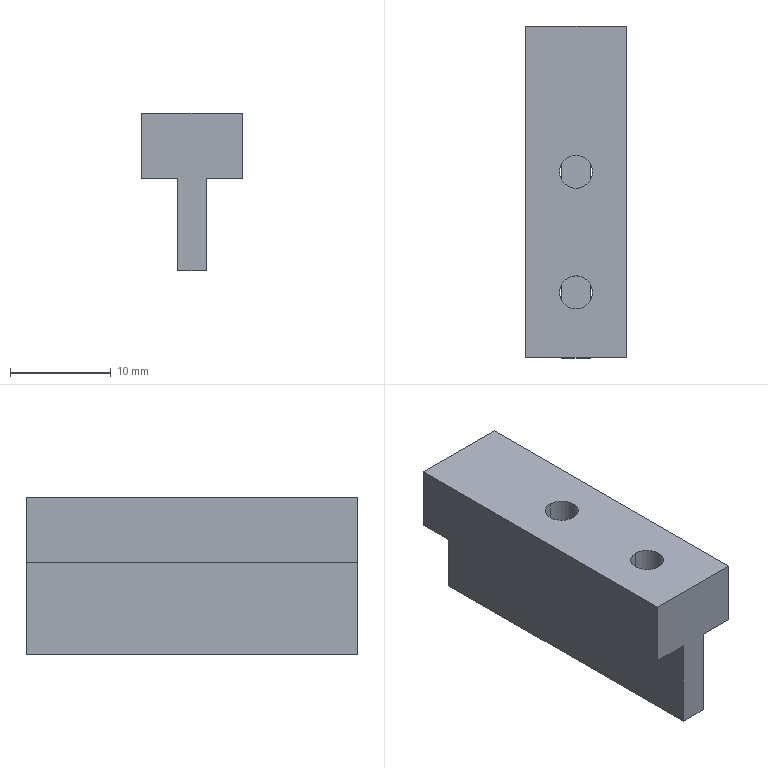Component | SolidWorks | 6G-TL06-X-AxisOrigin-1 | 1 solid | 16 faces | box 10 x 33 x 15.7 mm | volume 2884 mm3 | plane 12 | cylinder 4 | commonest cylinder face diameters 3.3 x4
build123d program:
from build123d import *

# Parameters (mm, degrees)
SKETCH1_W           = 33
SKETCH1_H           = 10
BOSS_EXTRUDE1_DEPTH = 6.5
M4_TAPPED_HOLE1_D   = 3.3
SKETCH7_W           = 33
SKETCH7_H           = 2.8
BOSS_EXTRUDE2_DEPTH = 9.2


with BuildPart() as part:
    # Sketch1 → Boss-Extrude1 (new body)
    with BuildSketch(Plane.XY):
        Rectangle(SKETCH1_W, SKETCH1_H)
    extrude(amount=-BOSS_EXTRUDE1_DEPTH)

    # M4 Tapped Hole1 (through all)
    with Locations(Plane(origin=(-10, 0, -6.5), x_dir=(-1, 0, 0), z_dir=(0, 0, -1))):
        with Locations((0, 0), (-12, 0)):
            Hole(M4_TAPPED_HOLE1_D / 2)

    # Sketch7 → Boss-Extrude2 (add)
    with BuildSketch(Plane(origin=(0, 0, -6.5), x_dir=(-1, 0, 0), z_dir=(0, 0, -1))):
        Rectangle(SKETCH7_W, SKETCH7_H)
    extrude(amount=BOSS_EXTRUDE2_DEPTH)


solid = part.part

# Placed as in the assembly
solid = solid.moved(Location((46, 333, -25), (0, 0, 90)))
STEP:
#1=COLOUR_RGB('',0.7922,0.8196,0.9333);
#2=FILL_AREA_STYLE_COLOUR('',#1);
#3=FILL_AREA_STYLE('',(#2));
#4=SURFACE_STYLE_FILL_AREA(#3);
#5=SURFACE_SIDE_STYLE('',(#4));
#6=SURFACE_STYLE_USAGE(.BOTH.,#5);
#7=PRESENTATION_STYLE_ASSIGNMENT((#6));
#8=CARTESIAN_POINT('',(1.811,12.781,-0.9843));
#9=VERTEX_POINT('',#8);
#10=CARTESIAN_POINT('',(1.811,12.652,-0.9843));
#11=VERTEX_POINT('',#10);
#12=CARTESIAN_POINT('',(1.811,12.717,-0.9843));
#13=DIRECTION('',(0.,-0.,-1.));
#14=DIRECTION('',(0.,-1.,0.));
#15=AXIS2_PLACEMENT_3D('',#12,#13,#14);
#16=CIRCLE('',#15,0.06496);
#17=EDGE_CURVE('',#9,#11,#16,.T.);
#18=ORIENTED_EDGE('',*,*,#17,.F.);
#19=CARTESIAN_POINT('',(1.811,12.781,-1.24));
#20=VERTEX_POINT('',#19);
#21=CARTESIAN_POINT('',(1.811,12.781,-1.24));
#22=DIRECTION('',(0.,-0.,-1.));
#23=VECTOR('',#22,39.37);
#24=LINE('',#21,#23);
#25=EDGE_CURVE('',#9,#20,#24,.T.);
#26=ORIENTED_EDGE('',*,*,#25,.T.);
#27=CARTESIAN_POINT('',(1.866,12.751,-1.24));
#28=VERTEX_POINT('',#27);
#29=CARTESIAN_POINT('',(1.811,12.717,-1.24));
#30=DIRECTION('',(0.,-0.,-1.));
#31=DIRECTION('',(0.,-1.,0.));
#32=AXIS2_PLACEMENT_3D('',#29,#30,#31);
#33=CIRCLE('',#32,0.06496);
#34=EDGE_CURVE('',#20,#28,#33,.T.);
#35=ORIENTED_EDGE('',*,*,#34,.T.);
#36=CARTESIAN_POINT('',(1.866,12.682,-1.24));
#37=VERTEX_POINT('',#36);
#38=CARTESIAN_POINT('',(1.811,12.717,-1.24));
#39=DIRECTION('',(0.,-0.,-1.));
#40=DIRECTION('',(0.,-1.,0.));
#41=AXIS2_PLACEMENT_3D('',#38,#39,#40);
#42=CIRCLE('',#41,0.06496);
#43=EDGE_CURVE('',#28,#37,#42,.T.);
#44=ORIENTED_EDGE('',*,*,#43,.T.);
#45=CARTESIAN_POINT('',(1.811,12.652,-1.24));
#46=VERTEX_POINT('',#45);
#47=CARTESIAN_POINT('',(1.811,12.717,-1.24));
#48=DIRECTION('',(0.,-0.,-1.));
#49=DIRECTION('',(0.,-1.,0.));
#50=AXIS2_PLACEMENT_3D('',#47,#48,#49);
#51=CIRCLE('',#50,0.06496);
#52=EDGE_CURVE('',#37,#46,#51,.T.);
#53=ORIENTED_EDGE('',*,*,#52,.T.);
#54=CARTESIAN_POINT('',(1.811,12.652,-1.24));
#55=DIRECTION('',(0.,-0.,-1.));
#56=VECTOR('',#55,39.37);
#57=LINE('',#54,#56);
#58=EDGE_CURVE('',#11,#46,#57,.T.);
#59=ORIENTED_EDGE('',*,*,#58,.F.);
#60=EDGE_LOOP('',(#18,#26,#35,#44,#53,#59));
#61=FACE_OUTER_BOUND('',#60,.T.);
#62=CARTESIAN_POINT('',(1.811,12.717,-1.24));
#63=DIRECTION('',(0.,-0.,-1.));
#64=DIRECTION('',(0.,-1.,0.));
#65=AXIS2_PLACEMENT_3D('',#62,#63,#64);
#66=CYLINDRICAL_SURFACE('',#65,0.06496);
#67=ADVANCED_FACE('',(#61),#66,.F.);
#68=CARTESIAN_POINT('',(1.811,13.254,-0.9843));
#69=VERTEX_POINT('',#68);
#70=CARTESIAN_POINT('',(1.811,13.124,-0.9843));
#71=VERTEX_POINT('',#70);
#72=CARTESIAN_POINT('',(1.811,13.189,-0.9843));
#73=DIRECTION('',(0.,-0.,-1.));
#74=DIRECTION('',(0.,-1.,0.));
#75=AXIS2_PLACEMENT_3D('',#72,#73,#74);
#76=CIRCLE('',#75,0.06496);
#77=EDGE_CURVE('',#69,#71,#76,.T.);
#78=ORIENTED_EDGE('',*,*,#77,.F.);
#79=CARTESIAN_POINT('',(1.811,13.254,-1.24));
#80=VERTEX_POINT('',#79);
#81=CARTESIAN_POINT('',(1.811,13.254,-1.24));
#82=DIRECTION('',(0.,-0.,-1.));
#83=VECTOR('',#82,39.37);
#84=LINE('',#81,#83);
#85=EDGE_CURVE('',#69,#80,#84,.T.);
#86=ORIENTED_EDGE('',*,*,#85,.T.);
#87=CARTESIAN_POINT('',(1.866,13.223,-1.24));
#88=VERTEX_POINT('',#87);
#89=CARTESIAN_POINT('',(1.811,13.189,-1.24));
#90=DIRECTION('',(0.,-0.,-1.));
#91=DIRECTION('',(0.,-1.,0.));
#92=AXIS2_PLACEMENT_3D('',#89,#90,#91);
#93=CIRCLE('',#92,0.06496);
#94=EDGE_CURVE('',#80,#88,#93,.T.);
#95=ORIENTED_EDGE('',*,*,#94,.T.);
#96=CARTESIAN_POINT('',(1.866,13.155,-1.24));
#97=VERTEX_POINT('',#96);
#98=CARTESIAN_POINT('',(1.811,13.189,-1.24));
#99=DIRECTION('',(0.,-0.,-1.));
#100=DIRECTION('',(0.,-1.,0.));
#101=AXIS2_PLACEMENT_3D('',#98,#99,#100);
#102=CIRCLE('',#101,0.06496);
#103=EDGE_CURVE('',#88,#97,#102,.T.);
#104=ORIENTED_EDGE('',*,*,#103,.T.);
#105=CARTESIAN_POINT('',(1.811,13.124,-1.24));
#106=VERTEX_POINT('',#105);
#107=CARTESIAN_POINT('',(1.811,13.189,-1.24));
#108=DIRECTION('',(0.,-0.,-1.));
#109=DIRECTION('',(0.,-1.,0.));
#110=AXIS2_PLACEMENT_3D('',#107,#108,#109);
#111=CIRCLE('',#110,0.06496);
#112=EDGE_CURVE('',#97,#106,#111,.T.);
#113=ORIENTED_EDGE('',*,*,#112,.T.);
#114=CARTESIAN_POINT('',(1.811,13.124,-1.24));
#115=DIRECTION('',(0.,-0.,-1.));
#116=VECTOR('',#115,39.37);
#117=LINE('',#114,#116);
#118=EDGE_CURVE('',#71,#106,#117,.T.);
#119=ORIENTED_EDGE('',*,*,#118,.F.);
#120=EDGE_LOOP('',(#78,#86,#95,#104,#113,#119));
#121=FACE_OUTER_BOUND('',#120,.T.);
#122=CARTESIAN_POINT('',(1.811,13.189,-1.24));
#123=DIRECTION('',(0.,-0.,-1.));
#124=DIRECTION('',(0.,-1.,0.));
#125=AXIS2_PLACEMENT_3D('',#122,#123,#124);
#126=CYLINDRICAL_SURFACE('',#125,0.06496);
#127=ADVANCED_FACE('',(#121),#126,.F.);
#128=CARTESIAN_POINT('',(1.866,13.76,-1.24));
#129=VERTEX_POINT('',#128);
#130=CARTESIAN_POINT('',(1.866,13.76,-1.24));
#131=DIRECTION('',(0.,-1.,0.));
#132=VECTOR('',#131,39.37);
#133=LINE('',#130,#132);
#134=EDGE_CURVE('',#129,#88,#133,.T.);
#135=ORIENTED_EDGE('',*,*,#134,.F.);
#136=CARTESIAN_POINT('',(2.008,13.76,-1.24));
#137=VERTEX_POINT('',#136);
#138=CARTESIAN_POINT('',(2.008,13.76,-1.24));
#139=DIRECTION('',(-1.,-0.,-0.));
#140=VECTOR('',#139,39.37);
#141=LINE('',#138,#140);
#142=EDGE_CURVE('',#137,#129,#141,.T.);
#143=ORIENTED_EDGE('',*,*,#142,.F.);
#144=CARTESIAN_POINT('',(2.008,12.461,-1.24));
#145=VERTEX_POINT('',#144);
#146=CARTESIAN_POINT('',(2.008,12.461,-1.24));
#147=DIRECTION('',(-0.,1.,-0.));
#148=VECTOR('',#147,39.37);
#149=LINE('',#146,#148);
#150=EDGE_CURVE('',#145,#137,#149,.T.);
#151=ORIENTED_EDGE('',*,*,#150,.F.);
#152=CARTESIAN_POINT('',(1.866,12.461,-1.24));
#153=VERTEX_POINT('',#152);
#154=CARTESIAN_POINT('',(2.008,12.461,-1.24));
#155=DIRECTION('',(1.,0.,0.));
#156=VECTOR('',#155,39.37);
#157=LINE('',#154,#156);
#158=EDGE_CURVE('',#153,#145,#157,.T.);
#159=ORIENTED_EDGE('',*,*,#158,.F.);
#160=CARTESIAN_POINT('',(1.866,13.76,-1.24));
#161=DIRECTION('',(0.,-1.,0.));
#162=VECTOR('',#161,39.37);
#163=LINE('',#160,#162);
#164=EDGE_CURVE('',#37,#153,#163,.T.);
#165=ORIENTED_EDGE('',*,*,#164,.F.);
#166=ORIENTED_EDGE('',*,*,#43,.F.);
#167=CARTESIAN_POINT('',(1.866,13.76,-1.24));
#168=DIRECTION('',(0.,-1.,0.));
#169=VECTOR('',#168,39.37);
#170=LINE('',#167,#169);
#171=EDGE_CURVE('',#97,#28,#170,.T.);
#172=ORIENTED_EDGE('',*,*,#171,.F.);
#173=ORIENTED_EDGE('',*,*,#103,.F.);
#174=EDGE_LOOP('',(#135,#143,#151,#159,#165,#166,#172,#173));
#175=FACE_OUTER_BOUND('',#174,.T.);
#176=CARTESIAN_POINT('',(1.811,13.11,-1.24));
#177=DIRECTION('',(0.,-0.,-1.));
#178=DIRECTION('',(0.,-1.,0.));
#179=AXIS2_PLACEMENT_3D('',#176,#177,#178);
#180=PLANE('',#179);
#181=ADVANCED_FACE('',(#175),#180,.T.);
#182=CARTESIAN_POINT('',(2.008,13.76,-0.9843));
#183=VERTEX_POINT('',#182);
#184=CARTESIAN_POINT('',(1.614,13.76,-0.9843));
#185=VERTEX_POINT('',#184);
#186=CARTESIAN_POINT('',(2.008,13.76,-0.9843));
#187=DIRECTION('',(-1.,-0.,-0.));
#188=VECTOR('',#187,39.37);
#189=LINE('',#186,#188);
#190=EDGE_CURVE('',#183,#185,#189,.T.);
#191=ORIENTED_EDGE('',*,*,#190,.F.);
#192=CARTESIAN_POINT('',(2.008,13.76,-1.24));
#193=DIRECTION('',(-0.,0.,1.));
#194=VECTOR('',#193,39.37);
#195=LINE('',#192,#194);
#196=EDGE_CURVE('',#137,#183,#195,.T.);
#197=ORIENTED_EDGE('',*,*,#196,.F.);
#198=ORIENTED_EDGE('',*,*,#142,.T.);
#199=CARTESIAN_POINT('',(1.866,13.76,-1.602));
#200=VERTEX_POINT('',#199);
#201=CARTESIAN_POINT('',(1.866,13.76,-1.602));
#202=DIRECTION('',(-0.,0.,1.));
#203=VECTOR('',#202,39.37);
#204=LINE('',#201,#203);
#205=EDGE_CURVE('',#200,#129,#204,.T.);
#206=ORIENTED_EDGE('',*,*,#205,.F.);
#207=CARTESIAN_POINT('',(1.756,13.76,-1.602));
#208=VERTEX_POINT('',#207);
#209=CARTESIAN_POINT('',(1.756,13.76,-1.602));
#210=DIRECTION('',(1.,0.,0.));
#211=VECTOR('',#210,39.37);
#212=LINE('',#209,#211);
#213=EDGE_CURVE('',#208,#200,#212,.T.);
#214=ORIENTED_EDGE('',*,*,#213,.F.);
#215=CARTESIAN_POINT('',(1.756,13.76,-1.24));
#216=VERTEX_POINT('',#215);
#217=CARTESIAN_POINT('',(1.756,13.76,-1.602));
#218=DIRECTION('',(-0.,0.,1.));
#219=VECTOR('',#218,39.37);
#220=LINE('',#217,#219);
#221=EDGE_CURVE('',#208,#216,#220,.T.);
#222=ORIENTED_EDGE('',*,*,#221,.T.);
#223=CARTESIAN_POINT('',(1.614,13.76,-1.24));
#224=VERTEX_POINT('',#223);
#225=CARTESIAN_POINT('',(2.008,13.76,-1.24));
#226=DIRECTION('',(-1.,-0.,-0.));
#227=VECTOR('',#226,39.37);
#228=LINE('',#225,#227);
#229=EDGE_CURVE('',#216,#224,#228,.T.);
#230=ORIENTED_EDGE('',*,*,#229,.T.);
#231=CARTESIAN_POINT('',(1.614,13.76,-1.24));
#232=DIRECTION('',(-0.,0.,1.));
#233=VECTOR('',#232,39.37);
#234=LINE('',#231,#233);
#235=EDGE_CURVE('',#224,#185,#234,.T.);
#236=ORIENTED_EDGE('',*,*,#235,.T.);
#237=EDGE_LOOP('',(#191,#197,#198,#206,#214,#222,#230,#236));
#238=FACE_OUTER_BOUND('',#237,.T.);
#239=CARTESIAN_POINT('',(2.008,13.76,-1.24));
#240=DIRECTION('',(-0.,1.,-0.));
#241=DIRECTION('',(0.,-0.,-1.));
#242=AXIS2_PLACEMENT_3D('',#239,#240,#241);
#243=PLANE('',#242);
#244=ADVANCED_FACE('',(#238),#243,.T.);
#245=CARTESIAN_POINT('',(2.008,12.461,-0.9843));
#246=VERTEX_POINT('',#245);
#247=CARTESIAN_POINT('',(2.008,12.461,-0.9843));
#248=DIRECTION('',(-0.,1.,-0.));
#249=VECTOR('',#248,39.37);
#250=LINE('',#247,#249);
#251=EDGE_CURVE('',#246,#183,#250,.T.);
#252=ORIENTED_EDGE('',*,*,#251,.F.);
#253=CARTESIAN_POINT('',(2.008,12.461,-1.24));
#254=DIRECTION('',(-0.,0.,1.));
#255=VECTOR('',#254,39.37);
#256=LINE('',#253,#255);
#257=EDGE_CURVE('',#145,#246,#256,.T.);
#258=ORIENTED_EDGE('',*,*,#257,.F.);
#259=ORIENTED_EDGE('',*,*,#150,.T.);
#260=ORIENTED_EDGE('',*,*,#196,.T.);
#261=EDGE_LOOP('',(#252,#258,#259,#260));
#262=FACE_OUTER_BOUND('',#261,.T.);
#263=CARTESIAN_POINT('',(2.008,12.461,-1.24));
#264=DIRECTION('',(1.,0.,0.));
#265=DIRECTION('',(0.,-0.,-1.));
#266=AXIS2_PLACEMENT_3D('',#263,#264,#265);
#267=PLANE('',#266);
#268=ADVANCED_FACE('',(#262),#267,.T.);
#269=CARTESIAN_POINT('',(1.614,12.461,-0.9843));
#270=VERTEX_POINT('',#269);
#271=CARTESIAN_POINT('',(2.008,12.461,-0.9843));
#272=DIRECTION('',(1.,0.,0.));
#273=VECTOR('',#272,39.37);
#274=LINE('',#271,#273);
#275=EDGE_CURVE('',#270,#246,#274,.T.);
#276=ORIENTED_EDGE('',*,*,#275,.F.);
#277=CARTESIAN_POINT('',(1.614,12.461,-1.24));
#278=VERTEX_POINT('',#277);
#279=CARTESIAN_POINT('',(1.614,12.461,-1.24));
#280=DIRECTION('',(-0.,0.,1.));
#281=VECTOR('',#280,39.37);
#282=LINE('',#279,#281);
#283=EDGE_CURVE('',#278,#270,#282,.T.);
#284=ORIENTED_EDGE('',*,*,#283,.F.);
#285=CARTESIAN_POINT('',(1.756,12.461,-1.24));
#286=VERTEX_POINT('',#285);
#287=CARTESIAN_POINT('',(2.008,12.461,-1.24));
#288=DIRECTION('',(1.,0.,0.));
#289=VECTOR('',#288,39.37);
#290=LINE('',#287,#289);
#291=EDGE_CURVE('',#278,#286,#290,.T.);
#292=ORIENTED_EDGE('',*,*,#291,.T.);
#293=CARTESIAN_POINT('',(1.756,12.461,-1.602));
#294=VERTEX_POINT('',#293);
#295=CARTESIAN_POINT('',(1.756,12.461,-1.602));
#296=DIRECTION('',(-0.,0.,1.));
#297=VECTOR('',#296,39.37);
#298=LINE('',#295,#297);
#299=EDGE_CURVE('',#294,#286,#298,.T.);
#300=ORIENTED_EDGE('',*,*,#299,.F.);
#301=CARTESIAN_POINT('',(1.866,12.461,-1.602));
#302=VERTEX_POINT('',#301);
#303=CARTESIAN_POINT('',(1.866,12.461,-1.602));
#304=DIRECTION('',(-1.,-0.,-0.));
#305=VECTOR('',#304,39.37);
#306=LINE('',#303,#305);
#307=EDGE_CURVE('',#302,#294,#306,.T.);
#308=ORIENTED_EDGE('',*,*,#307,.F.);
#309=CARTESIAN_POINT('',(1.866,12.461,-1.602));
#310=DIRECTION('',(-0.,0.,1.));
#311=VECTOR('',#310,39.37);
#312=LINE('',#309,#311);
#313=EDGE_CURVE('',#302,#153,#312,.T.);
#314=ORIENTED_EDGE('',*,*,#313,.T.);
#315=ORIENTED_EDGE('',*,*,#158,.T.);
#316=ORIENTED_EDGE('',*,*,#257,.T.);
#317=EDGE_LOOP('',(#276,#284,#292,#300,#308,#314,#315,#316));
#318=FACE_OUTER_BOUND('',#317,.T.);
#319=CARTESIAN_POINT('',(2.008,12.461,-1.24));
#320=DIRECTION('',(0.,-1.,0.));
#321=DIRECTION('',(-0.,0.,1.));
#322=AXIS2_PLACEMENT_3D('',#319,#320,#321);
#323=PLANE('',#322);
#324=ADVANCED_FACE('',(#318),#323,.T.);
#325=CARTESIAN_POINT('',(1.614,12.461,-0.9843));
#326=DIRECTION('',(0.,-1.,0.));
#327=VECTOR('',#326,39.37);
#328=LINE('',#325,#327);
#329=EDGE_CURVE('',#185,#270,#328,.T.);
#330=ORIENTED_EDGE('',*,*,#329,.F.);
#331=ORIENTED_EDGE('',*,*,#235,.F.);
#332=CARTESIAN_POINT('',(1.614,12.461,-1.24));
#333=DIRECTION('',(0.,-1.,0.));
#334=VECTOR('',#333,39.37);
#335=LINE('',#332,#334);
#336=EDGE_CURVE('',#224,#278,#335,.T.);
#337=ORIENTED_EDGE('',*,*,#336,.T.);
#338=ORIENTED_EDGE('',*,*,#283,.T.);
#339=EDGE_LOOP('',(#330,#331,#337,#338));
#340=FACE_OUTER_BOUND('',#339,.T.);
#341=CARTESIAN_POINT('',(1.614,12.461,-1.24));
#342=DIRECTION('',(-1.,-0.,-0.));
#343=DIRECTION('',(-0.,0.,1.));
#344=AXIS2_PLACEMENT_3D('',#341,#342,#343);
#345=PLANE('',#344);
#346=ADVANCED_FACE('',(#340),#345,.T.);
#347=CARTESIAN_POINT('',(1.756,12.682,-1.24));
#348=VERTEX_POINT('',#347);
#349=CARTESIAN_POINT('',(1.756,13.76,-1.24));
#350=DIRECTION('',(-0.,1.,-0.));
#351=VECTOR('',#350,39.37);
#352=LINE('',#349,#351);
#353=EDGE_CURVE('',#286,#348,#352,.T.);
#354=ORIENTED_EDGE('',*,*,#353,.F.);
#355=ORIENTED_EDGE('',*,*,#291,.F.);
#356=ORIENTED_EDGE('',*,*,#336,.F.);
#357=ORIENTED_EDGE('',*,*,#229,.F.);
#358=CARTESIAN_POINT('',(1.756,13.223,-1.24));
#359=VERTEX_POINT('',#358);
#360=CARTESIAN_POINT('',(1.756,13.76,-1.24));
#361=DIRECTION('',(-0.,1.,-0.));
#362=VECTOR('',#361,39.37);
#363=LINE('',#360,#362);
#364=EDGE_CURVE('',#359,#216,#363,.T.);
#365=ORIENTED_EDGE('',*,*,#364,.F.);
#366=CARTESIAN_POINT('',(1.756,13.155,-1.24));
#367=VERTEX_POINT('',#366);
#368=CARTESIAN_POINT('',(1.811,13.189,-1.24));
#369=DIRECTION('',(0.,-0.,-1.));
#370=DIRECTION('',(0.,-1.,0.));
#371=AXIS2_PLACEMENT_3D('',#368,#369,#370);
#372=CIRCLE('',#371,0.06496);
#373=EDGE_CURVE('',#367,#359,#372,.T.);
#374=ORIENTED_EDGE('',*,*,#373,.F.);
#375=CARTESIAN_POINT('',(1.756,12.751,-1.24));
#376=VERTEX_POINT('',#375);
#377=CARTESIAN_POINT('',(1.756,13.76,-1.24));
#378=DIRECTION('',(-0.,1.,-0.));
#379=VECTOR('',#378,39.37);
#380=LINE('',#377,#379);
#381=EDGE_CURVE('',#376,#367,#380,.T.);
#382=ORIENTED_EDGE('',*,*,#381,.F.);
#383=CARTESIAN_POINT('',(1.811,12.717,-1.24));
#384=DIRECTION('',(0.,-0.,-1.));
#385=DIRECTION('',(0.,-1.,0.));
#386=AXIS2_PLACEMENT_3D('',#383,#384,#385);
#387=CIRCLE('',#386,0.06496);
#388=EDGE_CURVE('',#348,#376,#387,.T.);
#389=ORIENTED_EDGE('',*,*,#388,.F.);
#390=EDGE_LOOP('',(#354,#355,#356,#357,#365,#374,#382,#389));
#391=FACE_OUTER_BOUND('',#390,.T.);
#392=CARTESIAN_POINT('',(1.811,13.11,-1.24));
#393=DIRECTION('',(0.,-0.,-1.));
#394=DIRECTION('',(0.,-1.,0.));
#395=AXIS2_PLACEMENT_3D('',#392,#393,#394);
#396=PLANE('',#395);
#397=ADVANCED_FACE('',(#391),#396,.T.);
#398=CARTESIAN_POINT('',(1.811,12.717,-0.9843));
#399=DIRECTION('',(0.,-0.,-1.));
#400=DIRECTION('',(0.,-1.,0.));
#401=AXIS2_PLACEMENT_3D('',#398,#399,#400);
#402=CIRCLE('',#401,0.06496);
#403=EDGE_CURVE('',#11,#9,#402,.T.);
#404=ORIENTED_EDGE('',*,*,#403,.T.);
#405=ORIENTED_EDGE('',*,*,#17,.T.);
#406=EDGE_LOOP('',(#404,#405));
#407=FACE_BOUND('',#406,.T.);
#408=CARTESIAN_POINT('',(1.811,13.189,-0.9843));
#409=DIRECTION('',(0.,-0.,-1.));
#410=DIRECTION('',(0.,-1.,0.));
#411=AXIS2_PLACEMENT_3D('',#408,#409,#410);
#412=CIRCLE('',#411,0.06496);
#413=EDGE_CURVE('',#71,#69,#412,.T.);
#414=ORIENTED_EDGE('',*,*,#413,.T.);
#415=ORIENTED_EDGE('',*,*,#77,.T.);
#416=EDGE_LOOP('',(#414,#415));
#417=FACE_BOUND('',#416,.T.);
#418=ORIENTED_EDGE('',*,*,#190,.T.);
#419=ORIENTED_EDGE('',*,*,#329,.T.);
#420=ORIENTED_EDGE('',*,*,#275,.T.);
#421=ORIENTED_EDGE('',*,*,#251,.T.);
#422=EDGE_LOOP('',(#418,#419,#420,#421));
#423=FACE_OUTER_BOUND('',#422,.T.);
#424=CARTESIAN_POINT('',(1.811,13.11,-0.9843));
#425=DIRECTION('',(0.,-0.,-1.));
#426=DIRECTION('',(0.,-1.,0.));
#427=AXIS2_PLACEMENT_3D('',#424,#425,#426);
#428=PLANE('',#427);
#429=ADVANCED_FACE('',(#407,#417,#423),#428,.F.);
#430=ORIENTED_EDGE('',*,*,#85,.F.);
#431=ORIENTED_EDGE('',*,*,#413,.F.);
#432=ORIENTED_EDGE('',*,*,#118,.T.);
#433=CARTESIAN_POINT('',(1.811,13.189,-1.24));
#434=DIRECTION('',(0.,-0.,-1.));
#435=DIRECTION('',(0.,-1.,0.));
#436=AXIS2_PLACEMENT_3D('',#433,#434,#435);
#437=CIRCLE('',#436,0.06496);
#438=EDGE_CURVE('',#106,#367,#437,.T.);
#439=ORIENTED_EDGE('',*,*,#438,.T.);
#440=ORIENTED_EDGE('',*,*,#373,.T.);
#441=CARTESIAN_POINT('',(1.811,13.189,-1.24));
#442=DIRECTION('',(0.,-0.,-1.));
#443=DIRECTION('',(0.,-1.,0.));
#444=AXIS2_PLACEMENT_3D('',#441,#442,#443);
#445=CIRCLE('',#444,0.06496);
#446=EDGE_CURVE('',#359,#80,#445,.T.);
#447=ORIENTED_EDGE('',*,*,#446,.T.);
#448=EDGE_LOOP('',(#430,#431,#432,#439,#440,#447));
#449=FACE_OUTER_BOUND('',#448,.T.);
#450=CARTESIAN_POINT('',(1.811,13.189,-1.24));
#451=DIRECTION('',(0.,-0.,-1.));
#452=DIRECTION('',(0.,-1.,0.));
#453=AXIS2_PLACEMENT_3D('',#450,#451,#452);
#454=CYLINDRICAL_SURFACE('',#453,0.06496);
#455=ADVANCED_FACE('',(#449),#454,.F.);
#456=ORIENTED_EDGE('',*,*,#25,.F.);
#457=ORIENTED_EDGE('',*,*,#403,.F.);
#458=ORIENTED_EDGE('',*,*,#58,.T.);
#459=CARTESIAN_POINT('',(1.811,12.717,-1.24));
#460=DIRECTION('',(0.,-0.,-1.));
#461=DIRECTION('',(0.,-1.,0.));
#462=AXIS2_PLACEMENT_3D('',#459,#460,#461);
#463=CIRCLE('',#462,0.06496);
#464=EDGE_CURVE('',#46,#348,#463,.T.);
#465=ORIENTED_EDGE('',*,*,#464,.T.);
#466=ORIENTED_EDGE('',*,*,#388,.T.);
#467=CARTESIAN_POINT('',(1.811,12.717,-1.24));
#468=DIRECTION('',(0.,-0.,-1.));
#469=DIRECTION('',(0.,-1.,0.));
#470=AXIS2_PLACEMENT_3D('',#467,#468,#469);
#471=CIRCLE('',#470,0.06496);
#472=EDGE_CURVE('',#376,#20,#471,.T.);
#473=ORIENTED_EDGE('',*,*,#472,.T.);
#474=EDGE_LOOP('',(#456,#457,#458,#465,#466,#473));
#475=FACE_OUTER_BOUND('',#474,.T.);
#476=CARTESIAN_POINT('',(1.811,12.717,-1.24));
#477=DIRECTION('',(0.,-0.,-1.));
#478=DIRECTION('',(0.,-1.,0.));
#479=AXIS2_PLACEMENT_3D('',#476,#477,#478);
#480=CYLINDRICAL_SURFACE('',#479,0.06496);
#481=ADVANCED_FACE('',(#475),#480,.F.);
#482=ORIENTED_EDGE('',*,*,#472,.F.);
#483=CARTESIAN_POINT('',(1.756,13.76,-1.24));
#484=DIRECTION('',(-0.,1.,-0.));
#485=VECTOR('',#484,39.37);
#486=LINE('',#483,#485);
#487=EDGE_CURVE('',#348,#376,#486,.T.);
#488=ORIENTED_EDGE('',*,*,#487,.F.);
#489=ORIENTED_EDGE('',*,*,#464,.F.);
#490=ORIENTED_EDGE('',*,*,#52,.F.);
#491=CARTESIAN_POINT('',(1.866,13.76,-1.24));
#492=DIRECTION('',(0.,-1.,0.));
#493=VECTOR('',#492,39.37);
#494=LINE('',#491,#493);
#495=EDGE_CURVE('',#28,#37,#494,.T.);
#496=ORIENTED_EDGE('',*,*,#495,.F.);
#497=ORIENTED_EDGE('',*,*,#34,.F.);
#498=EDGE_LOOP('',(#482,#488,#489,#490,#496,#497));
#499=FACE_OUTER_BOUND('',#498,.T.);
#500=CARTESIAN_POINT('',(1.811,13.11,-1.24));
#501=DIRECTION('',(-0.,0.,1.));
#502=DIRECTION('',(-0.,1.,-0.));
#503=AXIS2_PLACEMENT_3D('',#500,#501,#502);
#504=PLANE('',#503);
#505=ADVANCED_FACE('',(#499),#504,.T.);
#506=ORIENTED_EDGE('',*,*,#446,.F.);
#507=CARTESIAN_POINT('',(1.756,13.76,-1.24));
#508=DIRECTION('',(-0.,1.,-0.));
#509=VECTOR('',#508,39.37);
#510=LINE('',#507,#509);
#511=EDGE_CURVE('',#367,#359,#510,.T.);
#512=ORIENTED_EDGE('',*,*,#511,.F.);
#513=ORIENTED_EDGE('',*,*,#438,.F.);
#514=ORIENTED_EDGE('',*,*,#112,.F.);
#515=CARTESIAN_POINT('',(1.866,13.76,-1.24));
#516=DIRECTION('',(0.,-1.,0.));
#517=VECTOR('',#516,39.37);
#518=LINE('',#515,#517);
#519=EDGE_CURVE('',#88,#97,#518,.T.);
#520=ORIENTED_EDGE('',*,*,#519,.F.);
#521=ORIENTED_EDGE('',*,*,#94,.F.);
#522=EDGE_LOOP('',(#506,#512,#513,#514,#520,#521));
#523=FACE_OUTER_BOUND('',#522,.T.);
#524=CARTESIAN_POINT('',(1.811,13.11,-1.24));
#525=DIRECTION('',(-0.,0.,1.));
#526=DIRECTION('',(-0.,1.,-0.));
#527=AXIS2_PLACEMENT_3D('',#524,#525,#526);
#528=PLANE('',#527);
#529=ADVANCED_FACE('',(#523),#528,.T.);
#530=ORIENTED_EDGE('',*,*,#353,.T.);
#531=ORIENTED_EDGE('',*,*,#487,.T.);
#532=ORIENTED_EDGE('',*,*,#381,.T.);
#533=ORIENTED_EDGE('',*,*,#511,.T.);
#534=ORIENTED_EDGE('',*,*,#364,.T.);
#535=ORIENTED_EDGE('',*,*,#221,.F.);
#536=CARTESIAN_POINT('',(1.756,13.76,-1.602));
#537=DIRECTION('',(-0.,1.,-0.));
#538=VECTOR('',#537,39.37);
#539=LINE('',#536,#538);
#540=EDGE_CURVE('',#294,#208,#539,.T.);
#541=ORIENTED_EDGE('',*,*,#540,.F.);
#542=ORIENTED_EDGE('',*,*,#299,.T.);
#543=EDGE_LOOP('',(#530,#531,#532,#533,#534,#535,#541,#542));
#544=FACE_OUTER_BOUND('',#543,.T.);
#545=CARTESIAN_POINT('',(1.756,13.76,-1.602));
#546=DIRECTION('',(1.,0.,0.));
#547=DIRECTION('',(-0.,1.,-0.));
#548=AXIS2_PLACEMENT_3D('',#545,#546,#547);
#549=PLANE('',#548);
#550=ADVANCED_FACE('',(#544),#549,.F.);
#551=ORIENTED_EDGE('',*,*,#134,.T.);
#552=ORIENTED_EDGE('',*,*,#519,.T.);
#553=ORIENTED_EDGE('',*,*,#171,.T.);
#554=ORIENTED_EDGE('',*,*,#495,.T.);
#555=ORIENTED_EDGE('',*,*,#164,.T.);
#556=ORIENTED_EDGE('',*,*,#313,.F.);
#557=CARTESIAN_POINT('',(1.866,13.76,-1.602));
#558=DIRECTION('',(0.,-1.,0.));
#559=VECTOR('',#558,39.37);
#560=LINE('',#557,#559);
#561=EDGE_CURVE('',#200,#302,#560,.T.);
#562=ORIENTED_EDGE('',*,*,#561,.F.);
#563=ORIENTED_EDGE('',*,*,#205,.T.);
#564=EDGE_LOOP('',(#551,#552,#553,#554,#555,#556,#562,#563));
#565=FACE_OUTER_BOUND('',#564,.T.);
#566=CARTESIAN_POINT('',(1.866,13.76,-1.602));
#567=DIRECTION('',(-1.,-0.,-0.));
#568=DIRECTION('',(0.,-1.,0.));
#569=AXIS2_PLACEMENT_3D('',#566,#567,#568);
#570=PLANE('',#569);
#571=ADVANCED_FACE('',(#565),#570,.F.);
#572=ORIENTED_EDGE('',*,*,#307,.T.);
#573=ORIENTED_EDGE('',*,*,#540,.T.);
#574=ORIENTED_EDGE('',*,*,#213,.T.);
#575=ORIENTED_EDGE('',*,*,#561,.T.);
#576=EDGE_LOOP('',(#572,#573,#574,#575));
#577=FACE_OUTER_BOUND('',#576,.T.);
#578=CARTESIAN_POINT('',(1.811,13.11,-1.602));
#579=DIRECTION('',(-0.,0.,1.));
#580=DIRECTION('',(-0.,1.,-0.));
#581=AXIS2_PLACEMENT_3D('',#578,#579,#580);
#582=PLANE('',#581);
#583=ADVANCED_FACE('',(#577),#582,.F.);
#584=CLOSED_SHELL('',(#67,#127,#181,#244,#268,#324,#346,#397,#429,#455,#481,#505,#529,#550,#571,#583));
#585=MANIFOLD_SOLID_BREP('',#584);
#586=STYLED_ITEM('',(#7),#585);
#587=PRESENTATION_LAYER_ASSIGNMENT('','',(#586));
#588=(LENGTH_UNIT()NAMED_UNIT(*)SI_UNIT($,.METRE.));
#589=LENGTH_MEASURE_WITH_UNIT(LENGTH_MEASURE(0.0254),#588);
#590=DIMENSIONAL_EXPONENTS(1.,0.,0.,0.,0.,0.,0.);
#591=(CONVERSION_BASED_UNIT('',#589)LENGTH_UNIT()NAMED_UNIT(#590));
#592=UNCERTAINTY_MEASURE_WITH_UNIT(LENGTH_MEASURE(0.00001),#591,'','');
#593=(NAMED_UNIT(*)PLANE_ANGLE_UNIT()SI_UNIT($,.RADIAN.));
#594=(NAMED_UNIT(*)SI_UNIT($,.STERADIAN.)SOLID_ANGLE_UNIT());
#595=(GEOMETRIC_REPRESENTATION_CONTEXT(3)GLOBAL_UNCERTAINTY_ASSIGNED_CONTEXT((#592))GLOBAL_UNIT_ASSIGNED_CONTEXT((#591,#593,#594))REPRESENTATION_CONTEXT('',''));
#596=MECHANICAL_DESIGN_GEOMETRIC_PRESENTATION_REPRESENTATION('',(#586),#595);
#597=CARTESIAN_POINT('',(0.,0.,0.));
#598=DIRECTION('',(0.,0.,1.));
#599=DIRECTION('',(1.,0.,0.));
#600=AXIS2_PLACEMENT_3D('',#597,#598,#599);
#601=(LENGTH_UNIT()NAMED_UNIT(*)SI_UNIT($,.METRE.));
#602=LENGTH_MEASURE_WITH_UNIT(LENGTH_MEASURE(0.0254),#601);
#603=DIMENSIONAL_EXPONENTS(1.,0.,0.,0.,0.,0.,0.);
#604=(CONVERSION_BASED_UNIT('',#602)LENGTH_UNIT()NAMED_UNIT(#603));
#605=UNCERTAINTY_MEASURE_WITH_UNIT(LENGTH_MEASURE(0.00001),#604,'','');
#606=(NAMED_UNIT(*)PLANE_ANGLE_UNIT()SI_UNIT($,.RADIAN.));
#607=(NAMED_UNIT(*)SI_UNIT($,.STERADIAN.)SOLID_ANGLE_UNIT());
#608=(GEOMETRIC_REPRESENTATION_CONTEXT(3)GLOBAL_UNCERTAINTY_ASSIGNED_CONTEXT((#605))GLOBAL_UNIT_ASSIGNED_CONTEXT((#604,#606,#607))REPRESENTATION_CONTEXT('',''));
#609=ADVANCED_BREP_SHAPE_REPRESENTATION('',(#585,#600),#608);